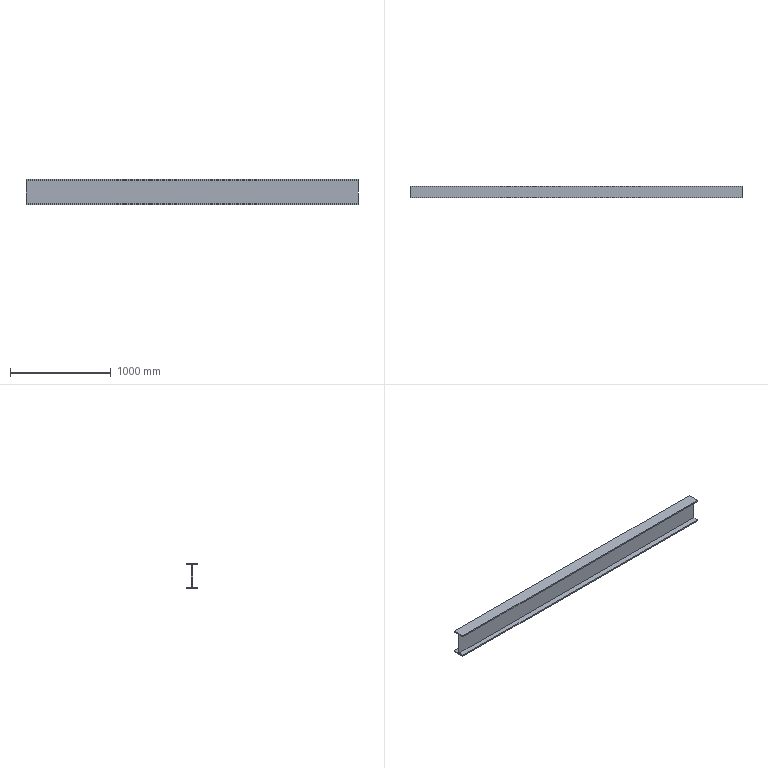Component | NX | CHUNSHUIJINCAO_1_11 | 1 solid | 14 faces | box 3300 x 118 x 250 mm | volume 17516400 mm3 | plane 14
STEP:
#1=CARTESIAN_POINT('',(0.,0.,0.));
#2=DIRECTION('',(0.,0.,1.));
#3=DIRECTION('',(1.,0.,0.));
#4=AXIS2_PLACEMENT_3D('',#1,#2,#3);
#5=CARTESIAN_POINT('',(3300.,6691.,250.));
#6=VERTEX_POINT('',#5);
#7=CARTESIAN_POINT('',(3300.,6809.,250.));
#8=VERTEX_POINT('',#7);
#9=CARTESIAN_POINT('',(3300.,6691.,250.));
#10=DIRECTION('',(0.,1.,0.));
#11=VECTOR('',#10,1.);
#12=LINE('',#9,#11);
#13=CARTESIAN_POINT('',(0.,6691.,250.));
#14=DIRECTION('',(0.,0.,-1.));
#15=DIRECTION('',(0.,-1.,-0.));
#16=AXIS2_PLACEMENT_3D('',#13,#14,#15);
#17=PLANE('',#16);
#18=CARTESIAN_POINT('',(0.,-3300.));
#19=DIRECTION('',(-1.,0.));
#20=VECTOR('',#19,1.);
#21=LINE('',#18,#20);
#22=(GEOMETRIC_REPRESENTATION_CONTEXT(2)PARAMETRIC_REPRESENTATION_CONTEXT()REPRESENTATION_CONTEXT('',''));
#23=DEFINITIONAL_REPRESENTATION('',(#21),#22);
#24=PCURVE('',#17,#23);
#25=CARTESIAN_POINT('',(3300.,6691.,250.));
#26=DIRECTION('',(-1.,0.,0.));
#27=DIRECTION('',(0.,0.,-1.));
#28=AXIS2_PLACEMENT_3D('',#25,#26,#27);
#29=PLANE('',#28);
#30=CARTESIAN_POINT('',(0.,0.));
#31=DIRECTION('',(-0.,-1.));
#32=VECTOR('',#31,1.);
#33=LINE('',#30,#32);
#34=(GEOMETRIC_REPRESENTATION_CONTEXT(2)PARAMETRIC_REPRESENTATION_CONTEXT()REPRESENTATION_CONTEXT('',''));
#35=DEFINITIONAL_REPRESENTATION('',(#33),#34);
#36=PCURVE('',#29,#35);
#37=SURFACE_CURVE('',#12,(#24,#36),.PCURVE_S1.);
#38=EDGE_CURVE('',#6,#8,#37,.T.);
#39=ORIENTED_EDGE('',*,*,#38,.T.);
#40=CARTESIAN_POINT('',(0.,6809.,250.));
#41=VERTEX_POINT('',#40);
#42=CARTESIAN_POINT('',(0.,6809.,250.));
#43=DIRECTION('',(1.,0.,0.));
#44=VECTOR('',#43,1.);
#45=LINE('',#42,#44);
#46=CARTESIAN_POINT('',(-118.,0.));
#47=DIRECTION('',(0.,-1.));
#48=VECTOR('',#47,1.);
#49=LINE('',#46,#48);
#50=(GEOMETRIC_REPRESENTATION_CONTEXT(2)PARAMETRIC_REPRESENTATION_CONTEXT()REPRESENTATION_CONTEXT('',''));
#51=DEFINITIONAL_REPRESENTATION('',(#49),#50);
#52=PCURVE('',#17,#51);
#53=CARTESIAN_POINT('',(0.,6809.,250.));
#54=DIRECTION('',(0.,-1.,0.));
#55=DIRECTION('',(-1.,0.,0.));
#56=AXIS2_PLACEMENT_3D('',#53,#54,#55);
#57=PLANE('',#56);
#58=CARTESIAN_POINT('',(0.,0.));
#59=DIRECTION('',(-1.,0.));
#60=VECTOR('',#59,1.);
#61=LINE('',#58,#60);
#62=(GEOMETRIC_REPRESENTATION_CONTEXT(2)PARAMETRIC_REPRESENTATION_CONTEXT()REPRESENTATION_CONTEXT('',''));
#63=DEFINITIONAL_REPRESENTATION('',(#61),#62);
#64=PCURVE('',#57,#63);
#65=SURFACE_CURVE('',#45,(#52,#64),.PCURVE_S1.);
#66=EDGE_CURVE('',#41,#8,#65,.T.);
#67=ORIENTED_EDGE('',*,*,#66,.F.);
#68=CARTESIAN_POINT('',(0.,6691.,250.));
#69=VERTEX_POINT('',#68);
#70=CARTESIAN_POINT('',(0.,6691.,250.));
#71=DIRECTION('',(0.,1.,0.));
#72=VECTOR('',#71,1.);
#73=LINE('',#70,#72);
#74=CARTESIAN_POINT('',(0.,0.));
#75=DIRECTION('',(-1.,0.));
#76=VECTOR('',#75,1.);
#77=LINE('',#74,#76);
#78=(GEOMETRIC_REPRESENTATION_CONTEXT(2)PARAMETRIC_REPRESENTATION_CONTEXT()REPRESENTATION_CONTEXT('',''));
#79=DEFINITIONAL_REPRESENTATION('',(#77),#78);
#80=PCURVE('',#17,#79);
#81=CARTESIAN_POINT('',(0.,6691.,250.));
#82=DIRECTION('',(-1.,0.,0.));
#83=DIRECTION('',(0.,0.,-1.));
#84=AXIS2_PLACEMENT_3D('',#81,#82,#83);
#85=PLANE('',#84);
#86=CARTESIAN_POINT('',(0.,0.));
#87=DIRECTION('',(-0.,-1.));
#88=VECTOR('',#87,1.);
#89=LINE('',#86,#88);
#90=(GEOMETRIC_REPRESENTATION_CONTEXT(2)PARAMETRIC_REPRESENTATION_CONTEXT()REPRESENTATION_CONTEXT('',''));
#91=DEFINITIONAL_REPRESENTATION('',(#89),#90);
#92=PCURVE('',#85,#91);
#93=SURFACE_CURVE('',#73,(#80,#92),.PCURVE_S1.);
#94=EDGE_CURVE('',#69,#41,#93,.T.);
#95=ORIENTED_EDGE('',*,*,#94,.F.);
#96=CARTESIAN_POINT('',(0.,6691.,250.));
#97=DIRECTION('',(1.,0.,0.));
#98=VECTOR('',#97,1.);
#99=LINE('',#96,#98);
#100=CARTESIAN_POINT('',(0.,0.));
#101=DIRECTION('',(0.,-1.));
#102=VECTOR('',#101,1.);
#103=LINE('',#100,#102);
#104=(GEOMETRIC_REPRESENTATION_CONTEXT(2)PARAMETRIC_REPRESENTATION_CONTEXT()REPRESENTATION_CONTEXT('',''));
#105=DEFINITIONAL_REPRESENTATION('',(#103),#104);
#106=PCURVE('',#17,#105);
#107=CARTESIAN_POINT('',(0.,6691.,237.));
#108=DIRECTION('',(0.,1.,0.));
#109=DIRECTION('',(1.,0.,0.));
#110=AXIS2_PLACEMENT_3D('',#107,#108,#109);
#111=PLANE('',#110);
#112=CARTESIAN_POINT('',(0.,-13.));
#113=DIRECTION('',(1.,0.));
#114=VECTOR('',#113,1.);
#115=LINE('',#112,#114);
#116=(GEOMETRIC_REPRESENTATION_CONTEXT(2)PARAMETRIC_REPRESENTATION_CONTEXT()REPRESENTATION_CONTEXT('',''));
#117=DEFINITIONAL_REPRESENTATION('',(#115),#116);
#118=PCURVE('',#111,#117);
#119=SURFACE_CURVE('',#99,(#106,#118),.PCURVE_S1.);
#120=EDGE_CURVE('',#69,#6,#119,.T.);
#121=ORIENTED_EDGE('',*,*,#120,.T.);
#122=EDGE_LOOP('',(#39,#67,#95,#121));
#123=FACE_BOUND('',#122,.T.);
#124=ADVANCED_FACE('',(#123),#17,.F.);
#125=CARTESIAN_POINT('',(3300.,6809.,237.));
#126=VERTEX_POINT('',#125);
#127=CARTESIAN_POINT('',(3300.,6809.,250.));
#128=DIRECTION('',(0.,0.,-1.));
#129=VECTOR('',#128,1.);
#130=LINE('',#127,#129);
#131=CARTESIAN_POINT('',(-3300.,0.));
#132=DIRECTION('',(0.,1.));
#133=VECTOR('',#132,1.);
#134=LINE('',#131,#133);
#135=(GEOMETRIC_REPRESENTATION_CONTEXT(2)PARAMETRIC_REPRESENTATION_CONTEXT()REPRESENTATION_CONTEXT('',''));
#136=DEFINITIONAL_REPRESENTATION('',(#134),#135);
#137=PCURVE('',#57,#136);
#138=CARTESIAN_POINT('',(0.,-118.));
#139=DIRECTION('',(1.,0.));
#140=VECTOR('',#139,1.);
#141=LINE('',#138,#140);
#142=(GEOMETRIC_REPRESENTATION_CONTEXT(2)PARAMETRIC_REPRESENTATION_CONTEXT()REPRESENTATION_CONTEXT('',''));
#143=DEFINITIONAL_REPRESENTATION('',(#141),#142);
#144=PCURVE('',#29,#143);
#145=SURFACE_CURVE('',#130,(#137,#144),.PCURVE_S1.);
#146=EDGE_CURVE('',#8,#126,#145,.T.);
#147=ORIENTED_EDGE('',*,*,#146,.T.);
#148=CARTESIAN_POINT('',(0.,6809.,237.));
#149=VERTEX_POINT('',#148);
#150=CARTESIAN_POINT('',(0.,6809.,237.));
#151=DIRECTION('',(1.,0.,0.));
#152=VECTOR('',#151,1.);
#153=LINE('',#150,#152);
#154=CARTESIAN_POINT('',(0.,13.));
#155=DIRECTION('',(-1.,0.));
#156=VECTOR('',#155,1.);
#157=LINE('',#154,#156);
#158=(GEOMETRIC_REPRESENTATION_CONTEXT(2)PARAMETRIC_REPRESENTATION_CONTEXT()REPRESENTATION_CONTEXT('',''));
#159=DEFINITIONAL_REPRESENTATION('',(#157),#158);
#160=PCURVE('',#57,#159);
#161=CARTESIAN_POINT('',(0.,6809.,237.));
#162=DIRECTION('',(0.,-0.,1.));
#163=DIRECTION('',(0.,1.,0.));
#164=AXIS2_PLACEMENT_3D('',#161,#162,#163);
#165=PLANE('',#164);
#166=CARTESIAN_POINT('',(0.,0.));
#167=DIRECTION('',(0.,-1.));
#168=VECTOR('',#167,1.);
#169=LINE('',#166,#168);
#170=(GEOMETRIC_REPRESENTATION_CONTEXT(2)PARAMETRIC_REPRESENTATION_CONTEXT()REPRESENTATION_CONTEXT('',''));
#171=DEFINITIONAL_REPRESENTATION('',(#169),#170);
#172=PCURVE('',#165,#171);
#173=SURFACE_CURVE('',#153,(#160,#172),.PCURVE_S1.);
#174=EDGE_CURVE('',#149,#126,#173,.T.);
#175=ORIENTED_EDGE('',*,*,#174,.F.);
#176=CARTESIAN_POINT('',(0.,6809.,250.));
#177=DIRECTION('',(0.,0.,-1.));
#178=VECTOR('',#177,1.);
#179=LINE('',#176,#178);
#180=CARTESIAN_POINT('',(0.,0.));
#181=DIRECTION('',(0.,1.));
#182=VECTOR('',#181,1.);
#183=LINE('',#180,#182);
#184=(GEOMETRIC_REPRESENTATION_CONTEXT(2)PARAMETRIC_REPRESENTATION_CONTEXT()REPRESENTATION_CONTEXT('',''));
#185=DEFINITIONAL_REPRESENTATION('',(#183),#184);
#186=PCURVE('',#57,#185);
#187=CARTESIAN_POINT('',(0.,-118.));
#188=DIRECTION('',(1.,0.));
#189=VECTOR('',#188,1.);
#190=LINE('',#187,#189);
#191=(GEOMETRIC_REPRESENTATION_CONTEXT(2)PARAMETRIC_REPRESENTATION_CONTEXT()REPRESENTATION_CONTEXT('',''));
#192=DEFINITIONAL_REPRESENTATION('',(#190),#191);
#193=PCURVE('',#85,#192);
#194=SURFACE_CURVE('',#179,(#186,#193),.PCURVE_S1.);
#195=EDGE_CURVE('',#41,#149,#194,.T.);
#196=ORIENTED_EDGE('',*,*,#195,.F.);
#197=ORIENTED_EDGE('',*,*,#66,.T.);
#198=EDGE_LOOP('',(#147,#175,#196,#197));
#199=FACE_BOUND('',#198,.T.);
#200=ADVANCED_FACE('',(#199),#57,.F.);
#201=CARTESIAN_POINT('',(3300.,6755.,237.));
#202=VERTEX_POINT('',#201);
#203=CARTESIAN_POINT('',(3300.,6809.,237.));
#204=DIRECTION('',(0.,-1.,-0.));
#205=VECTOR('',#204,1.);
#206=LINE('',#203,#205);
#207=CARTESIAN_POINT('',(0.,-3300.));
#208=DIRECTION('',(-1.,0.));
#209=VECTOR('',#208,1.);
#210=LINE('',#207,#209);
#211=(GEOMETRIC_REPRESENTATION_CONTEXT(2)PARAMETRIC_REPRESENTATION_CONTEXT()REPRESENTATION_CONTEXT('',''));
#212=DEFINITIONAL_REPRESENTATION('',(#210),#211);
#213=PCURVE('',#165,#212);
#214=CARTESIAN_POINT('',(13.,-118.));
#215=DIRECTION('',(0.,1.));
#216=VECTOR('',#215,1.);
#217=LINE('',#214,#216);
#218=(GEOMETRIC_REPRESENTATION_CONTEXT(2)PARAMETRIC_REPRESENTATION_CONTEXT()REPRESENTATION_CONTEXT('',''));
#219=DEFINITIONAL_REPRESENTATION('',(#217),#218);
#220=PCURVE('',#29,#219);
#221=SURFACE_CURVE('',#206,(#213,#220),.PCURVE_S1.);
#222=EDGE_CURVE('',#126,#202,#221,.T.);
#223=ORIENTED_EDGE('',*,*,#222,.T.);
#224=CARTESIAN_POINT('',(0.,6755.,237.));
#225=VERTEX_POINT('',#224);
#226=CARTESIAN_POINT('',(0.,6755.,237.));
#227=DIRECTION('',(1.,0.,0.));
#228=VECTOR('',#227,1.);
#229=LINE('',#226,#228);
#230=CARTESIAN_POINT('',(-54.,0.));
#231=DIRECTION('',(0.,-1.));
#232=VECTOR('',#231,1.);
#233=LINE('',#230,#232);
#234=(GEOMETRIC_REPRESENTATION_CONTEXT(2)PARAMETRIC_REPRESENTATION_CONTEXT()REPRESENTATION_CONTEXT('',''));
#235=DEFINITIONAL_REPRESENTATION('',(#233),#234);
#236=PCURVE('',#165,#235);
#237=CARTESIAN_POINT('',(0.,6755.,237.));
#238=DIRECTION('',(0.,-1.,-0.));
#239=DIRECTION('',(0.,-0.,1.));
#240=AXIS2_PLACEMENT_3D('',#237,#238,#239);
#241=PLANE('',#240);
#242=CARTESIAN_POINT('',(0.,0.));
#243=DIRECTION('',(0.,-1.));
#244=VECTOR('',#243,1.);
#245=LINE('',#242,#244);
#246=(GEOMETRIC_REPRESENTATION_CONTEXT(2)PARAMETRIC_REPRESENTATION_CONTEXT()REPRESENTATION_CONTEXT('',''));
#247=DEFINITIONAL_REPRESENTATION('',(#245),#246);
#248=PCURVE('',#241,#247);
#249=SURFACE_CURVE('',#229,(#236,#248),.PCURVE_S1.);
#250=EDGE_CURVE('',#225,#202,#249,.T.);
#251=ORIENTED_EDGE('',*,*,#250,.F.);
#252=CARTESIAN_POINT('',(0.,6809.,237.));
#253=DIRECTION('',(0.,-1.,-0.));
#254=VECTOR('',#253,1.);
#255=LINE('',#252,#254);
#256=CARTESIAN_POINT('',(0.,0.));
#257=DIRECTION('',(-1.,0.));
#258=VECTOR('',#257,1.);
#259=LINE('',#256,#258);
#260=(GEOMETRIC_REPRESENTATION_CONTEXT(2)PARAMETRIC_REPRESENTATION_CONTEXT()REPRESENTATION_CONTEXT('',''));
#261=DEFINITIONAL_REPRESENTATION('',(#259),#260);
#262=PCURVE('',#165,#261);
#263=CARTESIAN_POINT('',(13.,-118.));
#264=DIRECTION('',(0.,1.));
#265=VECTOR('',#264,1.);
#266=LINE('',#263,#265);
#267=(GEOMETRIC_REPRESENTATION_CONTEXT(2)PARAMETRIC_REPRESENTATION_CONTEXT()REPRESENTATION_CONTEXT('',''));
#268=DEFINITIONAL_REPRESENTATION('',(#266),#267);
#269=PCURVE('',#85,#268);
#270=SURFACE_CURVE('',#255,(#262,#269),.PCURVE_S1.);
#271=EDGE_CURVE('',#149,#225,#270,.T.);
#272=ORIENTED_EDGE('',*,*,#271,.F.);
#273=ORIENTED_EDGE('',*,*,#174,.T.);
#274=EDGE_LOOP('',(#223,#251,#272,#273));
#275=FACE_BOUND('',#274,.T.);
#276=ADVANCED_FACE('',(#275),#165,.F.);
#277=CARTESIAN_POINT('',(3300.,6755.,13.));
#278=VERTEX_POINT('',#277);
#279=CARTESIAN_POINT('',(3300.,6755.,237.));
#280=DIRECTION('',(0.,0.,-1.));
#281=VECTOR('',#280,1.);
#282=LINE('',#279,#281);
#283=CARTESIAN_POINT('',(0.,-3300.));
#284=DIRECTION('',(-1.,0.));
#285=VECTOR('',#284,1.);
#286=LINE('',#283,#285);
#287=(GEOMETRIC_REPRESENTATION_CONTEXT(2)PARAMETRIC_REPRESENTATION_CONTEXT()REPRESENTATION_CONTEXT('',''));
#288=DEFINITIONAL_REPRESENTATION('',(#286),#287);
#289=PCURVE('',#241,#288);
#290=CARTESIAN_POINT('',(13.,-64.));
#291=DIRECTION('',(1.,-0.));
#292=VECTOR('',#291,1.);
#293=LINE('',#290,#292);
#294=(GEOMETRIC_REPRESENTATION_CONTEXT(2)PARAMETRIC_REPRESENTATION_CONTEXT()REPRESENTATION_CONTEXT('',''));
#295=DEFINITIONAL_REPRESENTATION('',(#293),#294);
#296=PCURVE('',#29,#295);
#297=SURFACE_CURVE('',#282,(#289,#296),.PCURVE_S1.);
#298=EDGE_CURVE('',#202,#278,#297,.T.);
#299=ORIENTED_EDGE('',*,*,#298,.T.);
#300=CARTESIAN_POINT('',(0.,6755.,13.));
#301=VERTEX_POINT('',#300);
#302=CARTESIAN_POINT('',(0.,6755.,13.));
#303=DIRECTION('',(1.,0.,0.));
#304=VECTOR('',#303,1.);
#305=LINE('',#302,#304);
#306=CARTESIAN_POINT('',(-224.,0.));
#307=DIRECTION('',(0.,-1.));
#308=VECTOR('',#307,1.);
#309=LINE('',#306,#308);
#310=(GEOMETRIC_REPRESENTATION_CONTEXT(2)PARAMETRIC_REPRESENTATION_CONTEXT()REPRESENTATION_CONTEXT('',''));
#311=DEFINITIONAL_REPRESENTATION('',(#309),#310);
#312=PCURVE('',#241,#311);
#313=CARTESIAN_POINT('',(0.,6755.,13.));
#314=DIRECTION('',(0.,0.,-1.));
#315=DIRECTION('',(0.,-1.,-0.));
#316=AXIS2_PLACEMENT_3D('',#313,#314,#315);
#317=PLANE('',#316);
#318=CARTESIAN_POINT('',(0.,0.));
#319=DIRECTION('',(0.,-1.));
#320=VECTOR('',#319,1.);
#321=LINE('',#318,#320);
#322=(GEOMETRIC_REPRESENTATION_CONTEXT(2)PARAMETRIC_REPRESENTATION_CONTEXT()REPRESENTATION_CONTEXT('',''));
#323=DEFINITIONAL_REPRESENTATION('',(#321),#322);
#324=PCURVE('',#317,#323);
#325=SURFACE_CURVE('',#305,(#312,#324),.PCURVE_S1.);
#326=EDGE_CURVE('',#301,#278,#325,.T.);
#327=ORIENTED_EDGE('',*,*,#326,.F.);
#328=CARTESIAN_POINT('',(0.,6755.,237.));
#329=DIRECTION('',(0.,0.,-1.));
#330=VECTOR('',#329,1.);
#331=LINE('',#328,#330);
#332=CARTESIAN_POINT('',(0.,0.));
#333=DIRECTION('',(-1.,0.));
#334=VECTOR('',#333,1.);
#335=LINE('',#332,#334);
#336=(GEOMETRIC_REPRESENTATION_CONTEXT(2)PARAMETRIC_REPRESENTATION_CONTEXT()REPRESENTATION_CONTEXT('',''));
#337=DEFINITIONAL_REPRESENTATION('',(#335),#336);
#338=PCURVE('',#241,#337);
#339=CARTESIAN_POINT('',(13.,-64.));
#340=DIRECTION('',(1.,-0.));
#341=VECTOR('',#340,1.);
#342=LINE('',#339,#341);
#343=(GEOMETRIC_REPRESENTATION_CONTEXT(2)PARAMETRIC_REPRESENTATION_CONTEXT()REPRESENTATION_CONTEXT('',''));
#344=DEFINITIONAL_REPRESENTATION('',(#342),#343);
#345=PCURVE('',#85,#344);
#346=SURFACE_CURVE('',#331,(#338,#345),.PCURVE_S1.);
#347=EDGE_CURVE('',#225,#301,#346,.T.);
#348=ORIENTED_EDGE('',*,*,#347,.F.);
#349=ORIENTED_EDGE('',*,*,#250,.T.);
#350=EDGE_LOOP('',(#299,#327,#348,#349));
#351=FACE_BOUND('',#350,.T.);
#352=ADVANCED_FACE('',(#351),#241,.F.);
#353=CARTESIAN_POINT('',(3300.,6809.,13.));
#354=VERTEX_POINT('',#353);
#355=CARTESIAN_POINT('',(3300.,6755.,13.));
#356=DIRECTION('',(0.,1.,0.));
#357=VECTOR('',#356,1.);
#358=LINE('',#355,#357);
#359=CARTESIAN_POINT('',(0.,-3300.));
#360=DIRECTION('',(-1.,0.));
#361=VECTOR('',#360,1.);
#362=LINE('',#359,#361);
#363=(GEOMETRIC_REPRESENTATION_CONTEXT(2)PARAMETRIC_REPRESENTATION_CONTEXT()REPRESENTATION_CONTEXT('',''));
#364=DEFINITIONAL_REPRESENTATION('',(#362),#363);
#365=PCURVE('',#317,#364);
#366=CARTESIAN_POINT('',(237.,-64.));
#367=DIRECTION('',(-0.,-1.));
#368=VECTOR('',#367,1.);
#369=LINE('',#366,#368);
#370=(GEOMETRIC_REPRESENTATION_CONTEXT(2)PARAMETRIC_REPRESENTATION_CONTEXT()REPRESENTATION_CONTEXT('',''));
#371=DEFINITIONAL_REPRESENTATION('',(#369),#370);
#372=PCURVE('',#29,#371);
#373=SURFACE_CURVE('',#358,(#365,#372),.PCURVE_S1.);
#374=EDGE_CURVE('',#278,#354,#373,.T.);
#375=ORIENTED_EDGE('',*,*,#374,.T.);
#376=CARTESIAN_POINT('',(0.,6809.,13.));
#377=VERTEX_POINT('',#376);
#378=CARTESIAN_POINT('',(0.,6809.,13.));
#379=DIRECTION('',(1.,0.,0.));
#380=VECTOR('',#379,1.);
#381=LINE('',#378,#380);
#382=CARTESIAN_POINT('',(-54.,0.));
#383=DIRECTION('',(0.,-1.));
#384=VECTOR('',#383,1.);
#385=LINE('',#382,#384);
#386=(GEOMETRIC_REPRESENTATION_CONTEXT(2)PARAMETRIC_REPRESENTATION_CONTEXT()REPRESENTATION_CONTEXT('',''));
#387=DEFINITIONAL_REPRESENTATION('',(#385),#386);
#388=PCURVE('',#317,#387);
#389=CARTESIAN_POINT('',(0.,6809.,13.));
#390=DIRECTION('',(0.,-1.,-0.));
#391=DIRECTION('',(0.,-0.,1.));
#392=AXIS2_PLACEMENT_3D('',#389,#390,#391);
#393=PLANE('',#392);
#394=CARTESIAN_POINT('',(0.,0.));
#395=DIRECTION('',(0.,-1.));
#396=VECTOR('',#395,1.);
#397=LINE('',#394,#396);
#398=(GEOMETRIC_REPRESENTATION_CONTEXT(2)PARAMETRIC_REPRESENTATION_CONTEXT()REPRESENTATION_CONTEXT('',''));
#399=DEFINITIONAL_REPRESENTATION('',(#397),#398);
#400=PCURVE('',#393,#399);
#401=SURFACE_CURVE('',#381,(#388,#400),.PCURVE_S1.);
#402=EDGE_CURVE('',#377,#354,#401,.T.);
#403=ORIENTED_EDGE('',*,*,#402,.F.);
#404=CARTESIAN_POINT('',(0.,6755.,13.));
#405=DIRECTION('',(0.,1.,0.));
#406=VECTOR('',#405,1.);
#407=LINE('',#404,#406);
#408=CARTESIAN_POINT('',(0.,0.));
#409=DIRECTION('',(-1.,0.));
#410=VECTOR('',#409,1.);
#411=LINE('',#408,#410);
#412=(GEOMETRIC_REPRESENTATION_CONTEXT(2)PARAMETRIC_REPRESENTATION_CONTEXT()REPRESENTATION_CONTEXT('',''));
#413=DEFINITIONAL_REPRESENTATION('',(#411),#412);
#414=PCURVE('',#317,#413);
#415=CARTESIAN_POINT('',(237.,-64.));
#416=DIRECTION('',(-0.,-1.));
#417=VECTOR('',#416,1.);
#418=LINE('',#415,#417);
#419=(GEOMETRIC_REPRESENTATION_CONTEXT(2)PARAMETRIC_REPRESENTATION_CONTEXT()REPRESENTATION_CONTEXT('',''));
#420=DEFINITIONAL_REPRESENTATION('',(#418),#419);
#421=PCURVE('',#85,#420);
#422=SURFACE_CURVE('',#407,(#414,#421),.PCURVE_S1.);
#423=EDGE_CURVE('',#301,#377,#422,.T.);
#424=ORIENTED_EDGE('',*,*,#423,.F.);
#425=ORIENTED_EDGE('',*,*,#326,.T.);
#426=EDGE_LOOP('',(#375,#403,#424,#425));
#427=FACE_BOUND('',#426,.T.);
#428=ADVANCED_FACE('',(#427),#317,.F.);
#429=CARTESIAN_POINT('',(3300.,6809.,0.));
#430=VERTEX_POINT('',#429);
#431=CARTESIAN_POINT('',(3300.,6809.,13.));
#432=DIRECTION('',(0.,0.,-1.));
#433=VECTOR('',#432,1.);
#434=LINE('',#431,#433);
#435=CARTESIAN_POINT('',(0.,-3300.));
#436=DIRECTION('',(-1.,0.));
#437=VECTOR('',#436,1.);
#438=LINE('',#435,#437);
#439=(GEOMETRIC_REPRESENTATION_CONTEXT(2)PARAMETRIC_REPRESENTATION_CONTEXT()REPRESENTATION_CONTEXT('',''));
#440=DEFINITIONAL_REPRESENTATION('',(#438),#439);
#441=PCURVE('',#393,#440);
#442=CARTESIAN_POINT('',(237.,-118.));
#443=DIRECTION('',(1.,-0.));
#444=VECTOR('',#443,1.);
#445=LINE('',#442,#444);
#446=(GEOMETRIC_REPRESENTATION_CONTEXT(2)PARAMETRIC_REPRESENTATION_CONTEXT()REPRESENTATION_CONTEXT('',''));
#447=DEFINITIONAL_REPRESENTATION('',(#445),#446);
#448=PCURVE('',#29,#447);
#449=SURFACE_CURVE('',#434,(#441,#448),.PCURVE_S1.);
#450=EDGE_CURVE('',#354,#430,#449,.T.);
#451=ORIENTED_EDGE('',*,*,#450,.T.);
#452=CARTESIAN_POINT('',(0.,6809.,0.));
#453=VERTEX_POINT('',#452);
#454=CARTESIAN_POINT('',(0.,6809.,0.));
#455=DIRECTION('',(1.,0.,0.));
#456=VECTOR('',#455,1.);
#457=LINE('',#454,#456);
#458=CARTESIAN_POINT('',(-13.,0.));
#459=DIRECTION('',(0.,-1.));
#460=VECTOR('',#459,1.);
#461=LINE('',#458,#460);
#462=(GEOMETRIC_REPRESENTATION_CONTEXT(2)PARAMETRIC_REPRESENTATION_CONTEXT()REPRESENTATION_CONTEXT('',''));
#463=DEFINITIONAL_REPRESENTATION('',(#461),#462);
#464=PCURVE('',#393,#463);
#465=CARTESIAN_POINT('',(0.,6745.,0.));
#466=DIRECTION('',(0.,-0.,1.));
#467=DIRECTION('',(0.,1.,0.));
#468=AXIS2_PLACEMENT_3D('',#465,#466,#467);
#469=PLANE('',#468);
#470=CARTESIAN_POINT('',(64.,0.));
#471=DIRECTION('',(0.,-1.));
#472=VECTOR('',#471,1.);
#473=LINE('',#470,#472);
#474=(GEOMETRIC_REPRESENTATION_CONTEXT(2)PARAMETRIC_REPRESENTATION_CONTEXT()REPRESENTATION_CONTEXT('',''));
#475=DEFINITIONAL_REPRESENTATION('',(#473),#474);
#476=PCURVE('',#469,#475);
#477=SURFACE_CURVE('',#457,(#464,#476),.PCURVE_S1.);
#478=EDGE_CURVE('',#453,#430,#477,.T.);
#479=ORIENTED_EDGE('',*,*,#478,.F.);
#480=CARTESIAN_POINT('',(0.,6809.,13.));
#481=DIRECTION('',(0.,0.,-1.));
#482=VECTOR('',#481,1.);
#483=LINE('',#480,#482);
#484=CARTESIAN_POINT('',(0.,0.));
#485=DIRECTION('',(-1.,0.));
#486=VECTOR('',#485,1.);
#487=LINE('',#484,#486);
#488=(GEOMETRIC_REPRESENTATION_CONTEXT(2)PARAMETRIC_REPRESENTATION_CONTEXT()REPRESENTATION_CONTEXT('',''));
#489=DEFINITIONAL_REPRESENTATION('',(#487),#488);
#490=PCURVE('',#393,#489);
#491=CARTESIAN_POINT('',(237.,-118.));
#492=DIRECTION('',(1.,-0.));
#493=VECTOR('',#492,1.);
#494=LINE('',#491,#493);
#495=(GEOMETRIC_REPRESENTATION_CONTEXT(2)PARAMETRIC_REPRESENTATION_CONTEXT()REPRESENTATION_CONTEXT('',''));
#496=DEFINITIONAL_REPRESENTATION('',(#494),#495);
#497=PCURVE('',#85,#496);
#498=SURFACE_CURVE('',#483,(#490,#497),.PCURVE_S1.);
#499=EDGE_CURVE('',#377,#453,#498,.T.);
#500=ORIENTED_EDGE('',*,*,#499,.F.);
#501=ORIENTED_EDGE('',*,*,#402,.T.);
#502=EDGE_LOOP('',(#451,#479,#500,#501));
#503=FACE_BOUND('',#502,.T.);
#504=ADVANCED_FACE('',(#503),#393,.F.);
#505=CARTESIAN_POINT('',(3300.,6691.,0.));
#506=VERTEX_POINT('',#505);
#507=CARTESIAN_POINT('',(3300.,6745.,0.));
#508=DIRECTION('',(0.,-1.,-0.));
#509=VECTOR('',#508,1.);
#510=LINE('',#507,#509);
#511=CARTESIAN_POINT('',(0.,-3300.));
#512=DIRECTION('',(-1.,0.));
#513=VECTOR('',#512,1.);
#514=LINE('',#511,#513);
#515=(GEOMETRIC_REPRESENTATION_CONTEXT(2)PARAMETRIC_REPRESENTATION_CONTEXT()REPRESENTATION_CONTEXT('',''));
#516=DEFINITIONAL_REPRESENTATION('',(#514),#515);
#517=PCURVE('',#469,#516);
#518=CARTESIAN_POINT('',(250.,-54.));
#519=DIRECTION('',(0.,1.));
#520=VECTOR('',#519,1.);
#521=LINE('',#518,#520);
#522=(GEOMETRIC_REPRESENTATION_CONTEXT(2)PARAMETRIC_REPRESENTATION_CONTEXT()REPRESENTATION_CONTEXT('',''));
#523=DEFINITIONAL_REPRESENTATION('',(#521),#522);
#524=PCURVE('',#29,#523);
#525=SURFACE_CURVE('',#510,(#517,#524),.PCURVE_S1.);
#526=EDGE_CURVE('',#430,#506,#525,.T.);
#527=ORIENTED_EDGE('',*,*,#526,.T.);
#528=CARTESIAN_POINT('',(0.,6691.,0.));
#529=VERTEX_POINT('',#528);
#530=CARTESIAN_POINT('',(0.,6691.,0.));
#531=DIRECTION('',(1.,0.,0.));
#532=VECTOR('',#531,1.);
#533=LINE('',#530,#532);
#534=CARTESIAN_POINT('',(-54.,0.));
#535=DIRECTION('',(0.,-1.));
#536=VECTOR('',#535,1.);
#537=LINE('',#534,#536);
#538=(GEOMETRIC_REPRESENTATION_CONTEXT(2)PARAMETRIC_REPRESENTATION_CONTEXT()REPRESENTATION_CONTEXT('',''));
#539=DEFINITIONAL_REPRESENTATION('',(#537),#538);
#540=PCURVE('',#469,#539);
#541=CARTESIAN_POINT('',(0.,6691.,0.));
#542=DIRECTION('',(0.,1.,0.));
#543=DIRECTION('',(0.,0.,-1.));
#544=AXIS2_PLACEMENT_3D('',#541,#542,#543);
#545=PLANE('',#544);
#546=CARTESIAN_POINT('',(0.,0.));
#547=DIRECTION('',(0.,-1.));
#548=VECTOR('',#547,1.);
#549=LINE('',#546,#548);
#550=(GEOMETRIC_REPRESENTATION_CONTEXT(2)PARAMETRIC_REPRESENTATION_CONTEXT()REPRESENTATION_CONTEXT('',''));
#551=DEFINITIONAL_REPRESENTATION('',(#549),#550);
#552=PCURVE('',#545,#551);
#553=SURFACE_CURVE('',#533,(#540,#552),.PCURVE_S1.);
#554=EDGE_CURVE('',#529,#506,#553,.T.);
#555=ORIENTED_EDGE('',*,*,#554,.F.);
#556=CARTESIAN_POINT('',(0.,6809.,0.));
#557=DIRECTION('',(0.,-1.,-0.));
#558=VECTOR('',#557,1.);
#559=LINE('',#556,#558);
#560=CARTESIAN_POINT('',(64.,0.));
#561=DIRECTION('',(-1.,0.));
#562=VECTOR('',#561,1.);
#563=LINE('',#560,#562);
#564=(GEOMETRIC_REPRESENTATION_CONTEXT(2)PARAMETRIC_REPRESENTATION_CONTEXT()REPRESENTATION_CONTEXT('',''));
#565=DEFINITIONAL_REPRESENTATION('',(#563),#564);
#566=PCURVE('',#469,#565);
#567=CARTESIAN_POINT('',(250.,-118.));
#568=DIRECTION('',(0.,1.));
#569=VECTOR('',#568,1.);
#570=LINE('',#567,#569);
#571=(GEOMETRIC_REPRESENTATION_CONTEXT(2)PARAMETRIC_REPRESENTATION_CONTEXT()REPRESENTATION_CONTEXT('',''));
#572=DEFINITIONAL_REPRESENTATION('',(#570),#571);
#573=PCURVE('',#85,#572);
#574=SURFACE_CURVE('',#559,(#566,#573),.PCURVE_S1.);
#575=EDGE_CURVE('',#453,#529,#574,.T.);
#576=ORIENTED_EDGE('',*,*,#575,.F.);
#577=ORIENTED_EDGE('',*,*,#478,.T.);
#578=EDGE_LOOP('',(#527,#555,#576,#577));
#579=FACE_BOUND('',#578,.T.);
#580=ADVANCED_FACE('',(#579),#469,.F.);
#581=CARTESIAN_POINT('',(3300.,6691.,13.));
#582=VERTEX_POINT('',#581);
#583=CARTESIAN_POINT('',(3300.,6691.,0.));
#584=DIRECTION('',(0.,-0.,1.));
#585=VECTOR('',#584,1.);
#586=LINE('',#583,#585);
#587=CARTESIAN_POINT('',(0.,-3300.));
#588=DIRECTION('',(-1.,0.));
#589=VECTOR('',#588,1.);
#590=LINE('',#587,#589);
#591=(GEOMETRIC_REPRESENTATION_CONTEXT(2)PARAMETRIC_REPRESENTATION_CONTEXT()REPRESENTATION_CONTEXT('',''));
#592=DEFINITIONAL_REPRESENTATION('',(#590),#591);
#593=PCURVE('',#545,#592);
#594=CARTESIAN_POINT('',(250.,0.));
#595=DIRECTION('',(-1.,0.));
#596=VECTOR('',#595,1.);
#597=LINE('',#594,#596);
#598=(GEOMETRIC_REPRESENTATION_CONTEXT(2)PARAMETRIC_REPRESENTATION_CONTEXT()REPRESENTATION_CONTEXT('',''));
#599=DEFINITIONAL_REPRESENTATION('',(#597),#598);
#600=PCURVE('',#29,#599);
#601=SURFACE_CURVE('',#586,(#593,#600),.PCURVE_S1.);
#602=EDGE_CURVE('',#506,#582,#601,.T.);
#603=ORIENTED_EDGE('',*,*,#602,.T.);
#604=CARTESIAN_POINT('',(0.,6691.,13.));
#605=VERTEX_POINT('',#604);
#606=CARTESIAN_POINT('',(0.,6691.,13.));
#607=DIRECTION('',(1.,0.,0.));
#608=VECTOR('',#607,1.);
#609=LINE('',#606,#608);
#610=CARTESIAN_POINT('',(-13.,0.));
#611=DIRECTION('',(0.,-1.));
#612=VECTOR('',#611,1.);
#613=LINE('',#610,#612);
#614=(GEOMETRIC_REPRESENTATION_CONTEXT(2)PARAMETRIC_REPRESENTATION_CONTEXT()REPRESENTATION_CONTEXT('',''));
#615=DEFINITIONAL_REPRESENTATION('',(#613),#614);
#616=PCURVE('',#545,#615);
#617=CARTESIAN_POINT('',(0.,6691.,13.));
#618=DIRECTION('',(0.,0.,-1.));
#619=DIRECTION('',(0.,-1.,-0.));
#620=AXIS2_PLACEMENT_3D('',#617,#618,#619);
#621=PLANE('',#620);
#622=CARTESIAN_POINT('',(0.,0.));
#623=DIRECTION('',(0.,-1.));
#624=VECTOR('',#623,1.);
#625=LINE('',#622,#624);
#626=(GEOMETRIC_REPRESENTATION_CONTEXT(2)PARAMETRIC_REPRESENTATION_CONTEXT()REPRESENTATION_CONTEXT('',''));
#627=DEFINITIONAL_REPRESENTATION('',(#625),#626);
#628=PCURVE('',#621,#627);
#629=SURFACE_CURVE('',#609,(#616,#628),.PCURVE_S1.);
#630=EDGE_CURVE('',#605,#582,#629,.T.);
#631=ORIENTED_EDGE('',*,*,#630,.F.);
#632=CARTESIAN_POINT('',(0.,6691.,0.));
#633=DIRECTION('',(0.,-0.,1.));
#634=VECTOR('',#633,1.);
#635=LINE('',#632,#634);
#636=CARTESIAN_POINT('',(0.,0.));
#637=DIRECTION('',(-1.,0.));
#638=VECTOR('',#637,1.);
#639=LINE('',#636,#638);
#640=(GEOMETRIC_REPRESENTATION_CONTEXT(2)PARAMETRIC_REPRESENTATION_CONTEXT()REPRESENTATION_CONTEXT('',''));
#641=DEFINITIONAL_REPRESENTATION('',(#639),#640);
#642=PCURVE('',#545,#641);
#643=CARTESIAN_POINT('',(250.,0.));
#644=DIRECTION('',(-1.,0.));
#645=VECTOR('',#644,1.);
#646=LINE('',#643,#645);
#647=(GEOMETRIC_REPRESENTATION_CONTEXT(2)PARAMETRIC_REPRESENTATION_CONTEXT()REPRESENTATION_CONTEXT('',''));
#648=DEFINITIONAL_REPRESENTATION('',(#646),#647);
#649=PCURVE('',#85,#648);
#650=SURFACE_CURVE('',#635,(#642,#649),.PCURVE_S1.);
#651=EDGE_CURVE('',#529,#605,#650,.T.);
#652=ORIENTED_EDGE('',*,*,#651,.F.);
#653=ORIENTED_EDGE('',*,*,#554,.T.);
#654=EDGE_LOOP('',(#603,#631,#652,#653));
#655=FACE_BOUND('',#654,.T.);
#656=ADVANCED_FACE('',(#655),#545,.F.);
#657=CARTESIAN_POINT('',(3300.,6745.,13.));
#658=VERTEX_POINT('',#657);
#659=CARTESIAN_POINT('',(3300.,6691.,13.));
#660=DIRECTION('',(0.,1.,0.));
#661=VECTOR('',#660,1.);
#662=LINE('',#659,#661);
#663=CARTESIAN_POINT('',(0.,-3300.));
#664=DIRECTION('',(-1.,0.));
#665=VECTOR('',#664,1.);
#666=LINE('',#663,#665);
#667=(GEOMETRIC_REPRESENTATION_CONTEXT(2)PARAMETRIC_REPRESENTATION_CONTEXT()REPRESENTATION_CONTEXT('',''));
#668=DEFINITIONAL_REPRESENTATION('',(#666),#667);
#669=PCURVE('',#621,#668);
#670=CARTESIAN_POINT('',(237.,0.));
#671=DIRECTION('',(-0.,-1.));
#672=VECTOR('',#671,1.);
#673=LINE('',#670,#672);
#674=(GEOMETRIC_REPRESENTATION_CONTEXT(2)PARAMETRIC_REPRESENTATION_CONTEXT()REPRESENTATION_CONTEXT('',''));
#675=DEFINITIONAL_REPRESENTATION('',(#673),#674);
#676=PCURVE('',#29,#675);
#677=SURFACE_CURVE('',#662,(#669,#676),.PCURVE_S1.);
#678=EDGE_CURVE('',#582,#658,#677,.T.);
#679=ORIENTED_EDGE('',*,*,#678,.T.);
#680=CARTESIAN_POINT('',(0.,6745.,13.));
#681=VERTEX_POINT('',#680);
#682=CARTESIAN_POINT('',(0.,6745.,13.));
#683=DIRECTION('',(1.,0.,0.));
#684=VECTOR('',#683,1.);
#685=LINE('',#682,#684);
#686=CARTESIAN_POINT('',(-54.,0.));
#687=DIRECTION('',(0.,-1.));
#688=VECTOR('',#687,1.);
#689=LINE('',#686,#688);
#690=(GEOMETRIC_REPRESENTATION_CONTEXT(2)PARAMETRIC_REPRESENTATION_CONTEXT()REPRESENTATION_CONTEXT('',''));
#691=DEFINITIONAL_REPRESENTATION('',(#689),#690);
#692=PCURVE('',#621,#691);
#693=CARTESIAN_POINT('',(0.,6745.,13.));
#694=DIRECTION('',(0.,1.,0.));
#695=DIRECTION('',(0.,0.,-1.));
#696=AXIS2_PLACEMENT_3D('',#693,#694,#695);
#697=PLANE('',#696);
#698=CARTESIAN_POINT('',(0.,0.));
#699=DIRECTION('',(0.,-1.));
#700=VECTOR('',#699,1.);
#701=LINE('',#698,#700);
#702=(GEOMETRIC_REPRESENTATION_CONTEXT(2)PARAMETRIC_REPRESENTATION_CONTEXT()REPRESENTATION_CONTEXT('',''));
#703=DEFINITIONAL_REPRESENTATION('',(#701),#702);
#704=PCURVE('',#697,#703);
#705=SURFACE_CURVE('',#685,(#692,#704),.PCURVE_S1.);
#706=EDGE_CURVE('',#681,#658,#705,.T.);
#707=ORIENTED_EDGE('',*,*,#706,.F.);
#708=CARTESIAN_POINT('',(0.,6691.,13.));
#709=DIRECTION('',(0.,1.,0.));
#710=VECTOR('',#709,1.);
#711=LINE('',#708,#710);
#712=CARTESIAN_POINT('',(0.,0.));
#713=DIRECTION('',(-1.,0.));
#714=VECTOR('',#713,1.);
#715=LINE('',#712,#714);
#716=(GEOMETRIC_REPRESENTATION_CONTEXT(2)PARAMETRIC_REPRESENTATION_CONTEXT()REPRESENTATION_CONTEXT('',''));
#717=DEFINITIONAL_REPRESENTATION('',(#715),#716);
#718=PCURVE('',#621,#717);
#719=CARTESIAN_POINT('',(237.,0.));
#720=DIRECTION('',(-0.,-1.));
#721=VECTOR('',#720,1.);
#722=LINE('',#719,#721);
#723=(GEOMETRIC_REPRESENTATION_CONTEXT(2)PARAMETRIC_REPRESENTATION_CONTEXT()REPRESENTATION_CONTEXT('',''));
#724=DEFINITIONAL_REPRESENTATION('',(#722),#723);
#725=PCURVE('',#85,#724);
#726=SURFACE_CURVE('',#711,(#718,#725),.PCURVE_S1.);
#727=EDGE_CURVE('',#605,#681,#726,.T.);
#728=ORIENTED_EDGE('',*,*,#727,.F.);
#729=ORIENTED_EDGE('',*,*,#630,.T.);
#730=EDGE_LOOP('',(#679,#707,#728,#729));
#731=FACE_BOUND('',#730,.T.);
#732=ADVANCED_FACE('',(#731),#621,.F.);
#733=CARTESIAN_POINT('',(3300.,6745.,237.));
#734=VERTEX_POINT('',#733);
#735=CARTESIAN_POINT('',(3300.,6745.,13.));
#736=DIRECTION('',(0.,-0.,1.));
#737=VECTOR('',#736,1.);
#738=LINE('',#735,#737);
#739=CARTESIAN_POINT('',(0.,-3300.));
#740=DIRECTION('',(-1.,0.));
#741=VECTOR('',#740,1.);
#742=LINE('',#739,#741);
#743=(GEOMETRIC_REPRESENTATION_CONTEXT(2)PARAMETRIC_REPRESENTATION_CONTEXT()REPRESENTATION_CONTEXT('',''));
#744=DEFINITIONAL_REPRESENTATION('',(#742),#743);
#745=PCURVE('',#697,#744);
#746=CARTESIAN_POINT('',(237.,-54.));
#747=DIRECTION('',(-1.,0.));
#748=VECTOR('',#747,1.);
#749=LINE('',#746,#748);
#750=(GEOMETRIC_REPRESENTATION_CONTEXT(2)PARAMETRIC_REPRESENTATION_CONTEXT()REPRESENTATION_CONTEXT('',''));
#751=DEFINITIONAL_REPRESENTATION('',(#749),#750);
#752=PCURVE('',#29,#751);
#753=SURFACE_CURVE('',#738,(#745,#752),.PCURVE_S1.);
#754=EDGE_CURVE('',#658,#734,#753,.T.);
#755=ORIENTED_EDGE('',*,*,#754,.T.);
#756=CARTESIAN_POINT('',(0.,6745.,237.));
#757=VERTEX_POINT('',#756);
#758=CARTESIAN_POINT('',(0.,6745.,237.));
#759=DIRECTION('',(1.,0.,0.));
#760=VECTOR('',#759,1.);
#761=LINE('',#758,#760);
#762=CARTESIAN_POINT('',(-224.,0.));
#763=DIRECTION('',(0.,-1.));
#764=VECTOR('',#763,1.);
#765=LINE('',#762,#764);
#766=(GEOMETRIC_REPRESENTATION_CONTEXT(2)PARAMETRIC_REPRESENTATION_CONTEXT()REPRESENTATION_CONTEXT('',''));
#767=DEFINITIONAL_REPRESENTATION('',(#765),#766);
#768=PCURVE('',#697,#767);
#769=CARTESIAN_POINT('',(0.,6745.,237.));
#770=DIRECTION('',(0.,-0.,1.));
#771=DIRECTION('',(0.,1.,0.));
#772=AXIS2_PLACEMENT_3D('',#769,#770,#771);
#773=PLANE('',#772);
#774=CARTESIAN_POINT('',(0.,0.));
#775=DIRECTION('',(0.,-1.));
#776=VECTOR('',#775,1.);
#777=LINE('',#774,#776);
#778=(GEOMETRIC_REPRESENTATION_CONTEXT(2)PARAMETRIC_REPRESENTATION_CONTEXT()REPRESENTATION_CONTEXT('',''));
#779=DEFINITIONAL_REPRESENTATION('',(#777),#778);
#780=PCURVE('',#773,#779);
#781=SURFACE_CURVE('',#761,(#768,#780),.PCURVE_S1.);
#782=EDGE_CURVE('',#757,#734,#781,.T.);
#783=ORIENTED_EDGE('',*,*,#782,.F.);
#784=CARTESIAN_POINT('',(0.,6745.,13.));
#785=DIRECTION('',(0.,-0.,1.));
#786=VECTOR('',#785,1.);
#787=LINE('',#784,#786);
#788=CARTESIAN_POINT('',(0.,0.));
#789=DIRECTION('',(-1.,0.));
#790=VECTOR('',#789,1.);
#791=LINE('',#788,#790);
#792=(GEOMETRIC_REPRESENTATION_CONTEXT(2)PARAMETRIC_REPRESENTATION_CONTEXT()REPRESENTATION_CONTEXT('',''));
#793=DEFINITIONAL_REPRESENTATION('',(#791),#792);
#794=PCURVE('',#697,#793);
#795=CARTESIAN_POINT('',(237.,-54.));
#796=DIRECTION('',(-1.,0.));
#797=VECTOR('',#796,1.);
#798=LINE('',#795,#797);
#799=(GEOMETRIC_REPRESENTATION_CONTEXT(2)PARAMETRIC_REPRESENTATION_CONTEXT()REPRESENTATION_CONTEXT('',''));
#800=DEFINITIONAL_REPRESENTATION('',(#798),#799);
#801=PCURVE('',#85,#800);
#802=SURFACE_CURVE('',#787,(#794,#801),.PCURVE_S1.);
#803=EDGE_CURVE('',#681,#757,#802,.T.);
#804=ORIENTED_EDGE('',*,*,#803,.F.);
#805=ORIENTED_EDGE('',*,*,#706,.T.);
#806=EDGE_LOOP('',(#755,#783,#804,#805));
#807=FACE_BOUND('',#806,.T.);
#808=ADVANCED_FACE('',(#807),#697,.F.);
#809=CARTESIAN_POINT('',(3300.,6691.,237.));
#810=VERTEX_POINT('',#809);
#811=CARTESIAN_POINT('',(3300.,6745.,237.));
#812=DIRECTION('',(0.,-1.,-0.));
#813=VECTOR('',#812,1.);
#814=LINE('',#811,#813);
#815=CARTESIAN_POINT('',(0.,-3300.));
#816=DIRECTION('',(-1.,0.));
#817=VECTOR('',#816,1.);
#818=LINE('',#815,#817);
#819=(GEOMETRIC_REPRESENTATION_CONTEXT(2)PARAMETRIC_REPRESENTATION_CONTEXT()REPRESENTATION_CONTEXT('',''));
#820=DEFINITIONAL_REPRESENTATION('',(#818),#819);
#821=PCURVE('',#773,#820);
#822=CARTESIAN_POINT('',(13.,-54.));
#823=DIRECTION('',(0.,1.));
#824=VECTOR('',#823,1.);
#825=LINE('',#822,#824);
#826=(GEOMETRIC_REPRESENTATION_CONTEXT(2)PARAMETRIC_REPRESENTATION_CONTEXT()REPRESENTATION_CONTEXT('',''));
#827=DEFINITIONAL_REPRESENTATION('',(#825),#826);
#828=PCURVE('',#29,#827);
#829=SURFACE_CURVE('',#814,(#821,#828),.PCURVE_S1.);
#830=EDGE_CURVE('',#734,#810,#829,.T.);
#831=ORIENTED_EDGE('',*,*,#830,.T.);
#832=CARTESIAN_POINT('',(0.,6691.,237.));
#833=VERTEX_POINT('',#832);
#834=CARTESIAN_POINT('',(0.,6691.,237.));
#835=DIRECTION('',(1.,0.,0.));
#836=VECTOR('',#835,1.);
#837=LINE('',#834,#836);
#838=CARTESIAN_POINT('',(-54.,0.));
#839=DIRECTION('',(0.,-1.));
#840=VECTOR('',#839,1.);
#841=LINE('',#838,#840);
#842=(GEOMETRIC_REPRESENTATION_CONTEXT(2)PARAMETRIC_REPRESENTATION_CONTEXT()REPRESENTATION_CONTEXT('',''));
#843=DEFINITIONAL_REPRESENTATION('',(#841),#842);
#844=PCURVE('',#773,#843);
#845=CARTESIAN_POINT('',(0.,0.));
#846=DIRECTION('',(1.,0.));
#847=VECTOR('',#846,1.);
#848=LINE('',#845,#847);
#849=(GEOMETRIC_REPRESENTATION_CONTEXT(2)PARAMETRIC_REPRESENTATION_CONTEXT()REPRESENTATION_CONTEXT('',''));
#850=DEFINITIONAL_REPRESENTATION('',(#848),#849);
#851=PCURVE('',#111,#850);
#852=SURFACE_CURVE('',#837,(#844,#851),.PCURVE_S1.);
#853=EDGE_CURVE('',#833,#810,#852,.T.);
#854=ORIENTED_EDGE('',*,*,#853,.F.);
#855=CARTESIAN_POINT('',(0.,6745.,237.));
#856=DIRECTION('',(0.,-1.,-0.));
#857=VECTOR('',#856,1.);
#858=LINE('',#855,#857);
#859=CARTESIAN_POINT('',(0.,0.));
#860=DIRECTION('',(-1.,0.));
#861=VECTOR('',#860,1.);
#862=LINE('',#859,#861);
#863=(GEOMETRIC_REPRESENTATION_CONTEXT(2)PARAMETRIC_REPRESENTATION_CONTEXT()REPRESENTATION_CONTEXT('',''));
#864=DEFINITIONAL_REPRESENTATION('',(#862),#863);
#865=PCURVE('',#773,#864);
#866=CARTESIAN_POINT('',(13.,-54.));
#867=DIRECTION('',(0.,1.));
#868=VECTOR('',#867,1.);
#869=LINE('',#866,#868);
#870=(GEOMETRIC_REPRESENTATION_CONTEXT(2)PARAMETRIC_REPRESENTATION_CONTEXT()REPRESENTATION_CONTEXT('',''));
#871=DEFINITIONAL_REPRESENTATION('',(#869),#870);
#872=PCURVE('',#85,#871);
#873=SURFACE_CURVE('',#858,(#865,#872),.PCURVE_S1.);
#874=EDGE_CURVE('',#757,#833,#873,.T.);
#875=ORIENTED_EDGE('',*,*,#874,.F.);
#876=ORIENTED_EDGE('',*,*,#782,.T.);
#877=EDGE_LOOP('',(#831,#854,#875,#876));
#878=FACE_BOUND('',#877,.T.);
#879=ADVANCED_FACE('',(#878),#773,.F.);
#880=CARTESIAN_POINT('',(3300.,6691.,237.));
#881=DIRECTION('',(0.,0.,1.));
#882=VECTOR('',#881,1.);
#883=LINE('',#880,#882);
#884=CARTESIAN_POINT('',(3300.,0.));
#885=DIRECTION('',(0.,-1.));
#886=VECTOR('',#885,1.);
#887=LINE('',#884,#886);
#888=(GEOMETRIC_REPRESENTATION_CONTEXT(2)PARAMETRIC_REPRESENTATION_CONTEXT()REPRESENTATION_CONTEXT('',''));
#889=DEFINITIONAL_REPRESENTATION('',(#887),#888);
#890=PCURVE('',#111,#889);
#891=CARTESIAN_POINT('',(13.,0.));
#892=DIRECTION('',(-1.,0.));
#893=VECTOR('',#892,1.);
#894=LINE('',#891,#893);
#895=(GEOMETRIC_REPRESENTATION_CONTEXT(2)PARAMETRIC_REPRESENTATION_CONTEXT()REPRESENTATION_CONTEXT('',''));
#896=DEFINITIONAL_REPRESENTATION('',(#894),#895);
#897=PCURVE('',#29,#896);
#898=SURFACE_CURVE('',#883,(#890,#897),.PCURVE_S1.);
#899=EDGE_CURVE('',#810,#6,#898,.T.);
#900=ORIENTED_EDGE('',*,*,#899,.T.);
#901=ORIENTED_EDGE('',*,*,#120,.F.);
#902=CARTESIAN_POINT('',(0.,6691.,237.));
#903=DIRECTION('',(0.,0.,1.));
#904=VECTOR('',#903,1.);
#905=LINE('',#902,#904);
#906=CARTESIAN_POINT('',(0.,0.));
#907=DIRECTION('',(0.,-1.));
#908=VECTOR('',#907,1.);
#909=LINE('',#906,#908);
#910=(GEOMETRIC_REPRESENTATION_CONTEXT(2)PARAMETRIC_REPRESENTATION_CONTEXT()REPRESENTATION_CONTEXT('',''));
#911=DEFINITIONAL_REPRESENTATION('',(#909),#910);
#912=PCURVE('',#111,#911);
#913=CARTESIAN_POINT('',(13.,0.));
#914=DIRECTION('',(-1.,0.));
#915=VECTOR('',#914,1.);
#916=LINE('',#913,#915);
#917=(GEOMETRIC_REPRESENTATION_CONTEXT(2)PARAMETRIC_REPRESENTATION_CONTEXT()REPRESENTATION_CONTEXT('',''));
#918=DEFINITIONAL_REPRESENTATION('',(#916),#917);
#919=PCURVE('',#85,#918);
#920=SURFACE_CURVE('',#905,(#912,#919),.PCURVE_S1.);
#921=EDGE_CURVE('',#833,#69,#920,.T.);
#922=ORIENTED_EDGE('',*,*,#921,.F.);
#923=ORIENTED_EDGE('',*,*,#853,.T.);
#924=EDGE_LOOP('',(#900,#901,#922,#923));
#925=FACE_BOUND('',#924,.T.);
#926=ADVANCED_FACE('',(#925),#111,.F.);
#927=ORIENTED_EDGE('',*,*,#94,.T.);
#928=ORIENTED_EDGE('',*,*,#195,.T.);
#929=ORIENTED_EDGE('',*,*,#271,.T.);
#930=ORIENTED_EDGE('',*,*,#347,.T.);
#931=ORIENTED_EDGE('',*,*,#423,.T.);
#932=ORIENTED_EDGE('',*,*,#499,.T.);
#933=ORIENTED_EDGE('',*,*,#575,.T.);
#934=ORIENTED_EDGE('',*,*,#651,.T.);
#935=ORIENTED_EDGE('',*,*,#727,.T.);
#936=ORIENTED_EDGE('',*,*,#803,.T.);
#937=ORIENTED_EDGE('',*,*,#874,.T.);
#938=ORIENTED_EDGE('',*,*,#921,.T.);
#939=EDGE_LOOP('',(#927,#928,#929,#930,#931,#932,#933,#934,#935,#936,#937,#938));
#940=FACE_BOUND('',#939,.T.);
#941=ADVANCED_FACE('',(#940),#85,.T.);
#942=ORIENTED_EDGE('',*,*,#38,.F.);
#943=ORIENTED_EDGE('',*,*,#899,.F.);
#944=ORIENTED_EDGE('',*,*,#830,.F.);
#945=ORIENTED_EDGE('',*,*,#754,.F.);
#946=ORIENTED_EDGE('',*,*,#678,.F.);
#947=ORIENTED_EDGE('',*,*,#602,.F.);
#948=ORIENTED_EDGE('',*,*,#526,.F.);
#949=ORIENTED_EDGE('',*,*,#450,.F.);
#950=ORIENTED_EDGE('',*,*,#374,.F.);
#951=ORIENTED_EDGE('',*,*,#298,.F.);
#952=ORIENTED_EDGE('',*,*,#222,.F.);
#953=ORIENTED_EDGE('',*,*,#146,.F.);
#954=EDGE_LOOP('',(#942,#943,#944,#945,#946,#947,#948,#949,#950,#951,#952,#953));
#955=FACE_BOUND('',#954,.T.);
#956=ADVANCED_FACE('',(#955),#29,.F.);
#957=CLOSED_SHELL('',(#124,#200,#276,#352,#428,#504,#580,#656,#732,#808,#879,#926,#941,#956));
#958=MANIFOLD_SOLID_BREP('',#957);
#959=(LENGTH_UNIT()NAMED_UNIT(*)SI_UNIT(.MILLI.,.METRE.));
#960=UNCERTAINTY_MEASURE_WITH_UNIT(LENGTH_MEASURE(0.0000001),#959,'','');
#961=(NAMED_UNIT(*)PLANE_ANGLE_UNIT()SI_UNIT($,.RADIAN.));
#962=(NAMED_UNIT(*)SI_UNIT($,.STERADIAN.)SOLID_ANGLE_UNIT());
#963=(GEOMETRIC_REPRESENTATION_CONTEXT(3)GLOBAL_UNCERTAINTY_ASSIGNED_CONTEXT((#960))GLOBAL_UNIT_ASSIGNED_CONTEXT((#959,#961,#962))REPRESENTATION_CONTEXT('',''));
#964=ADVANCED_BREP_SHAPE_REPRESENTATION('',(#4,#958),#963);